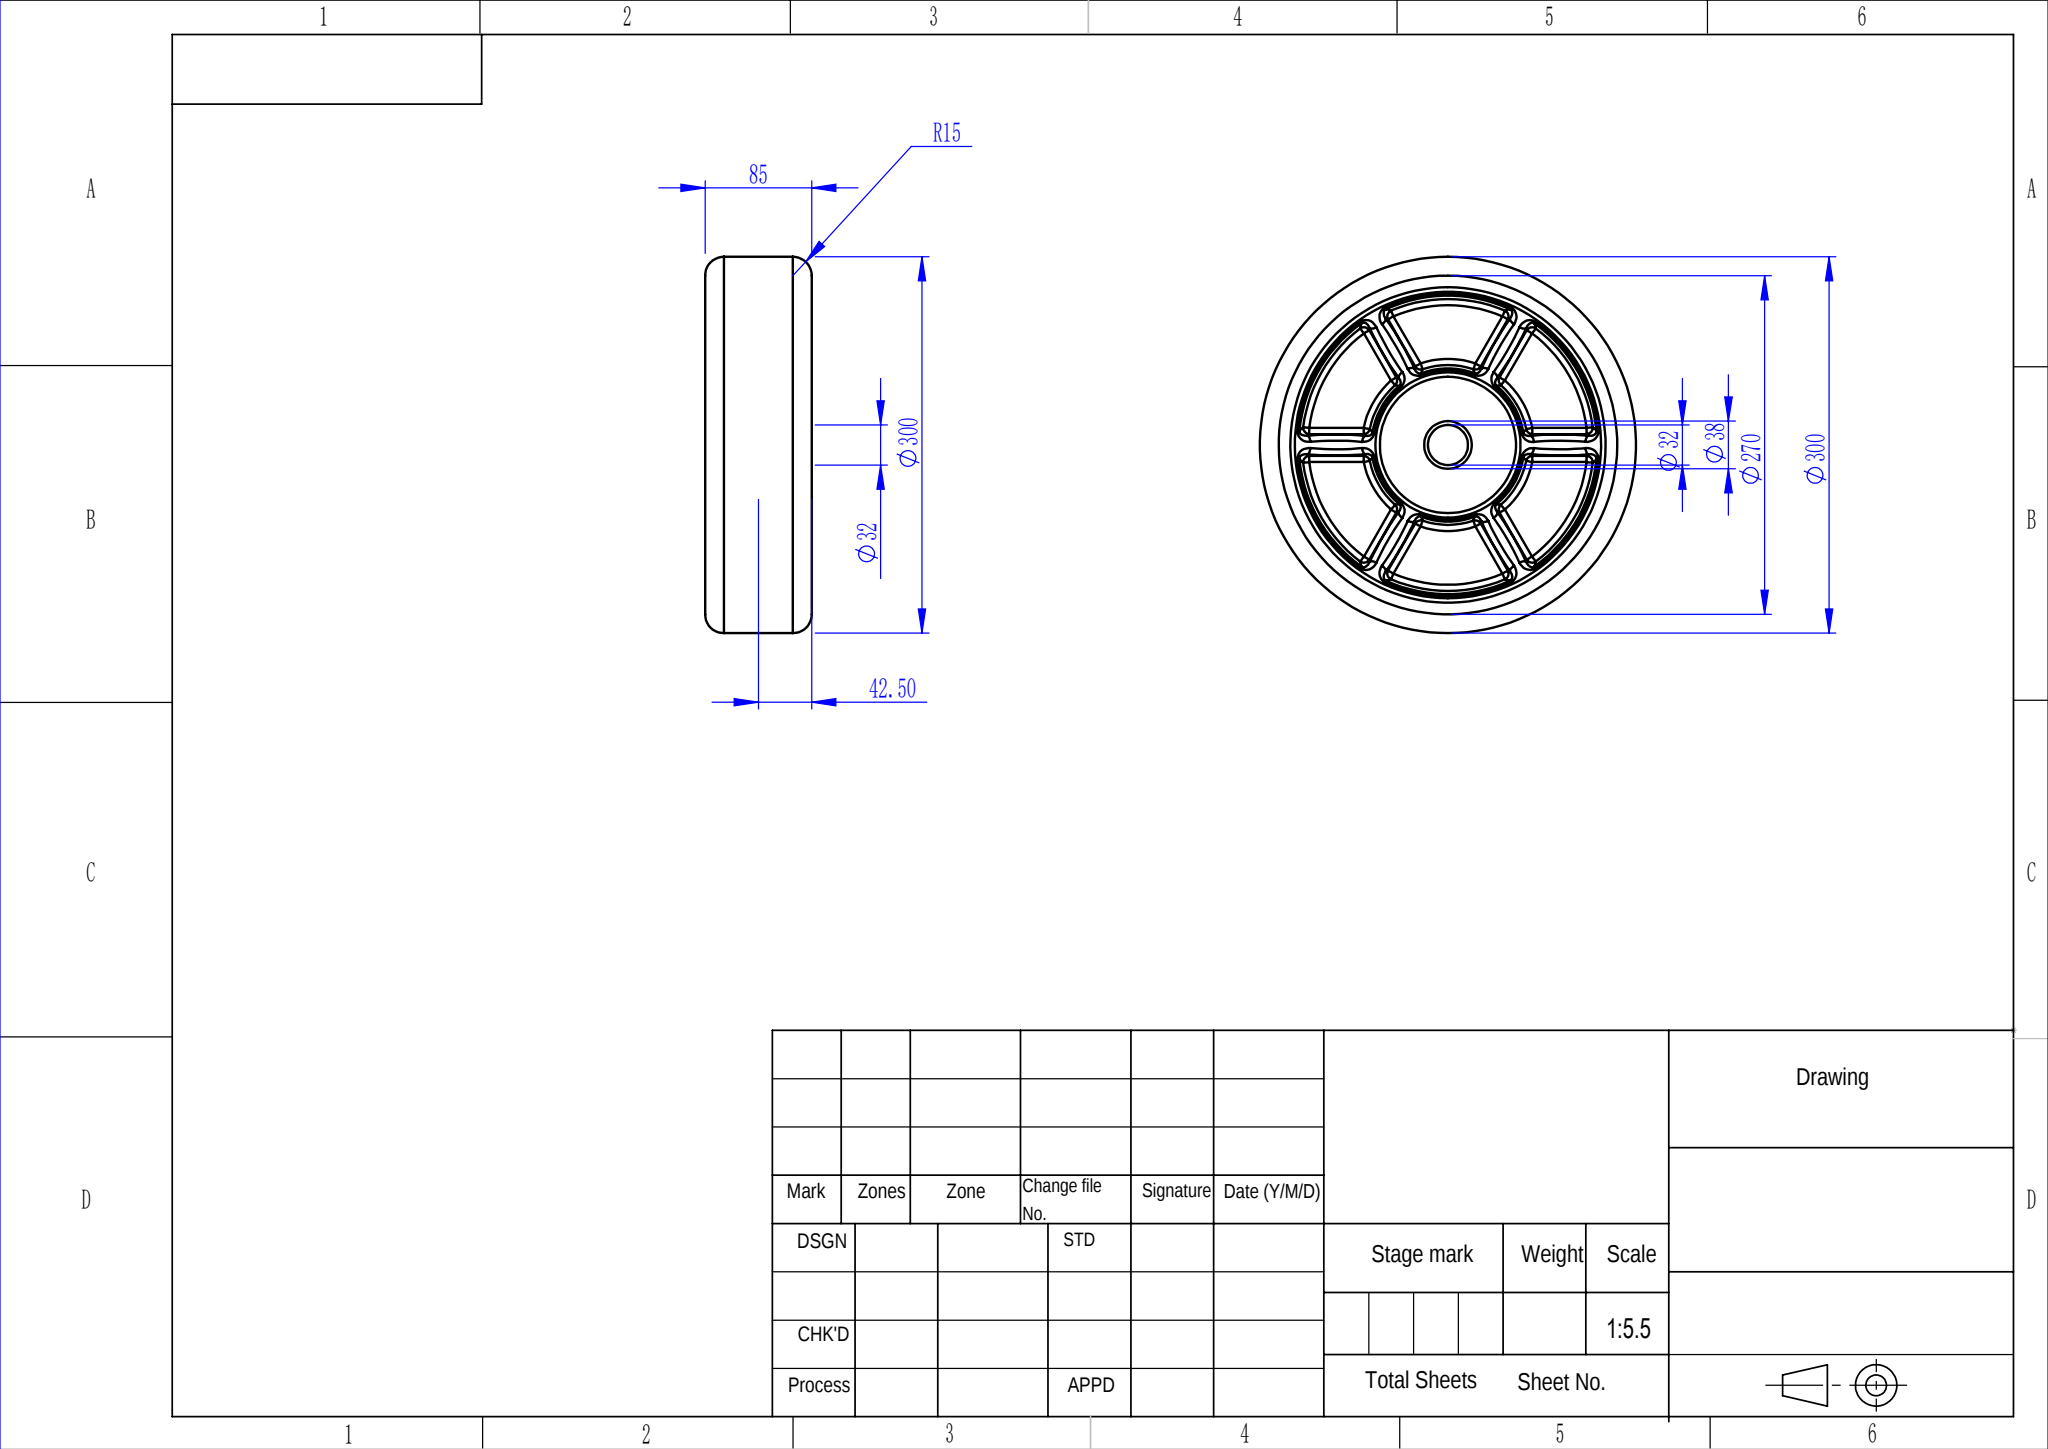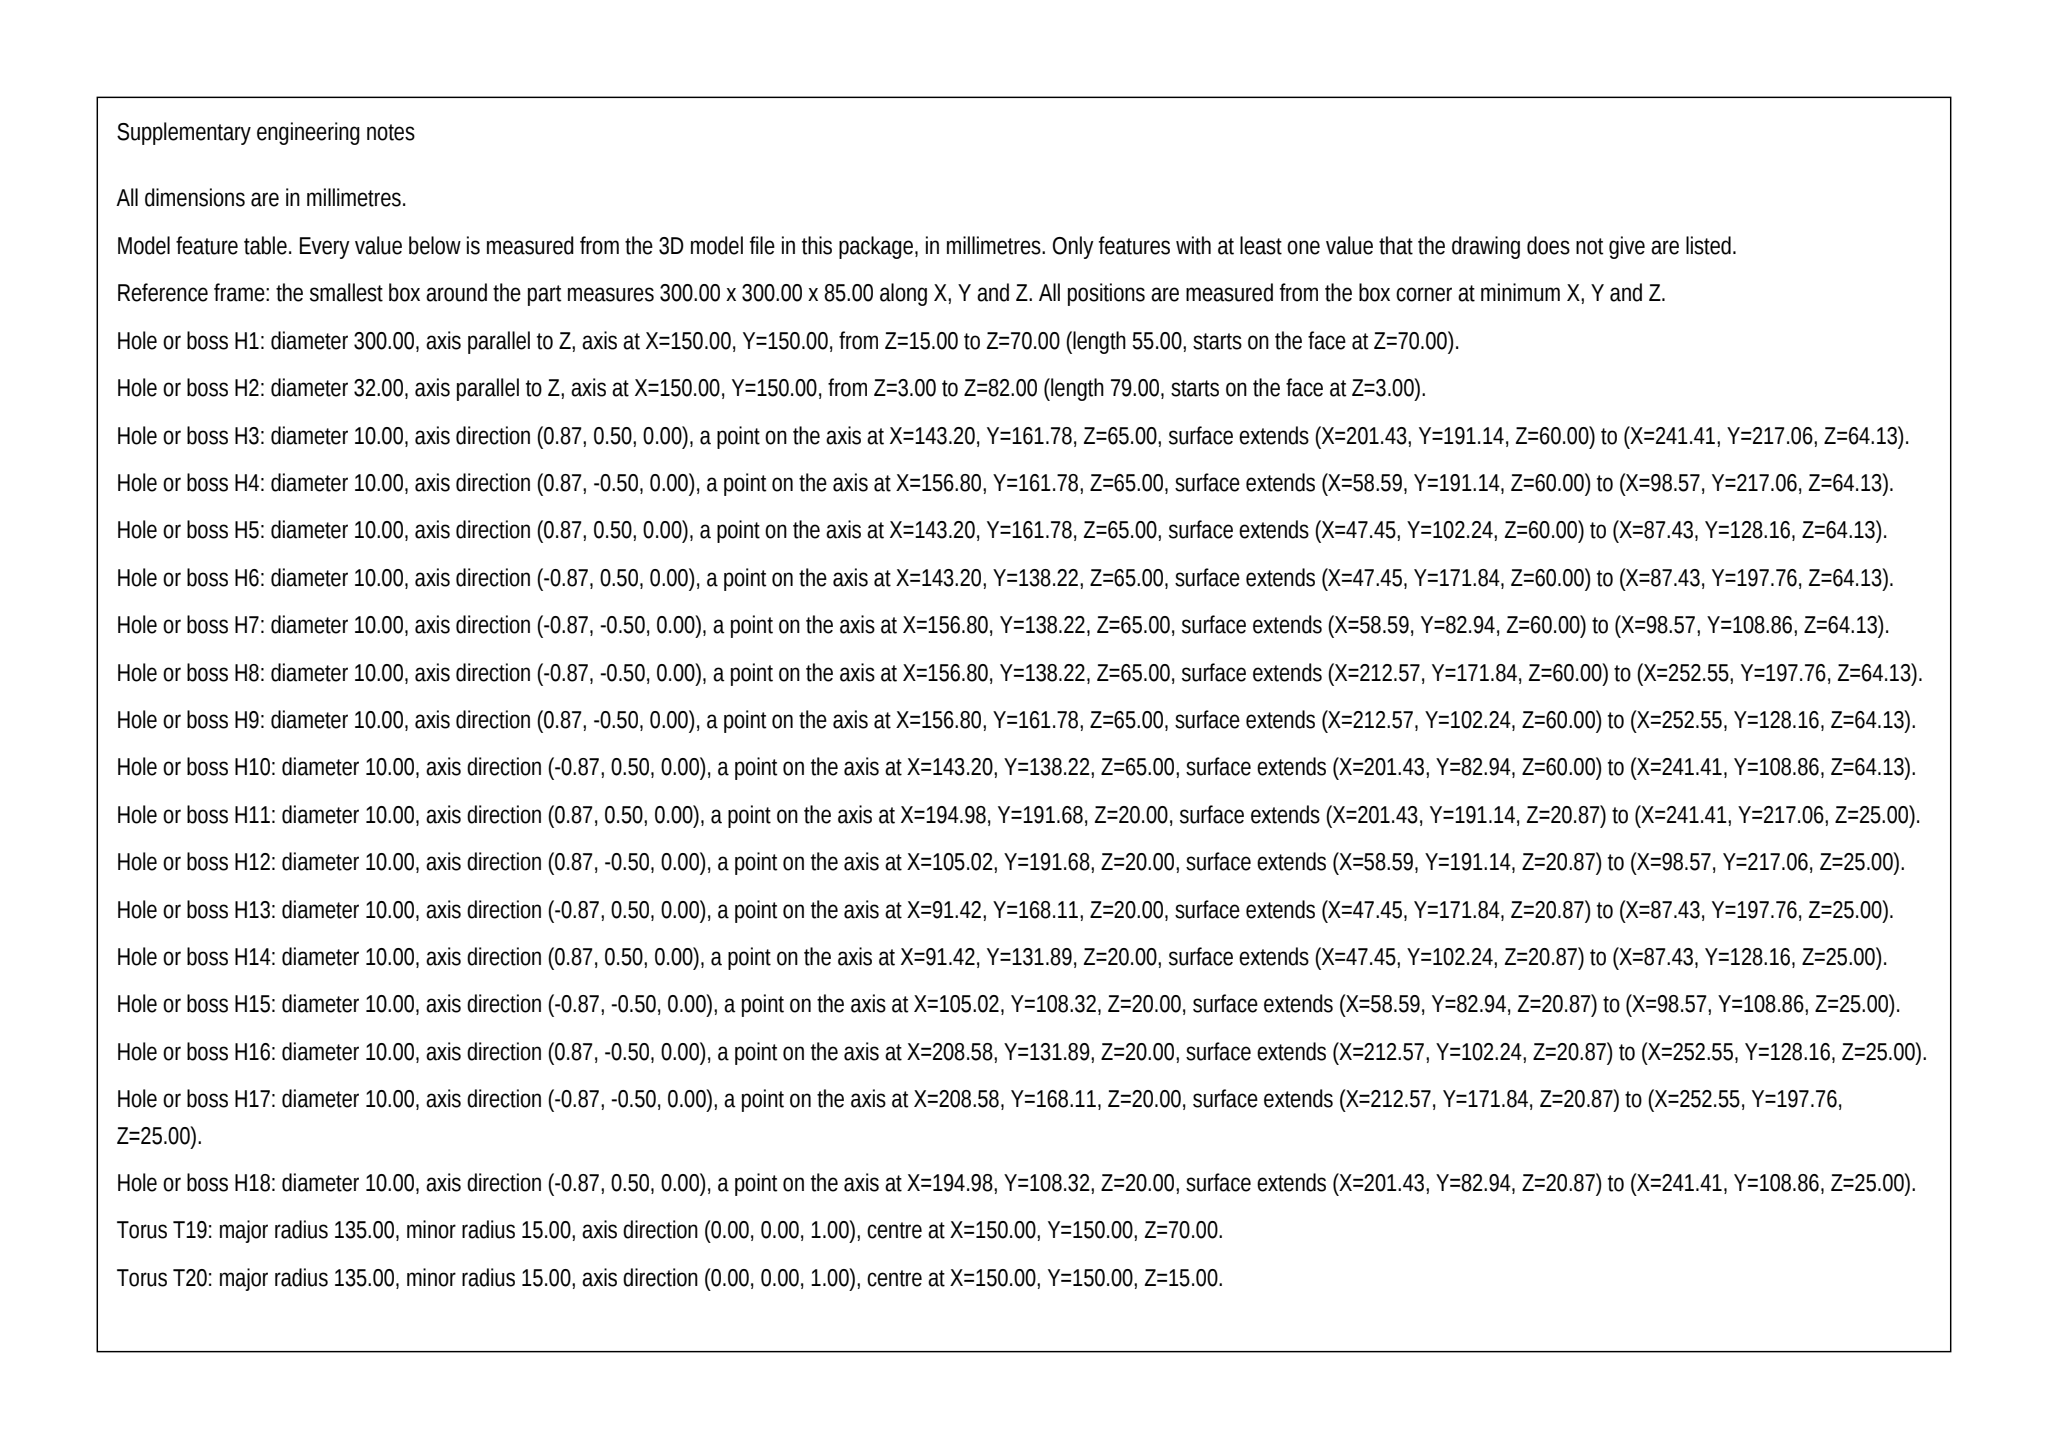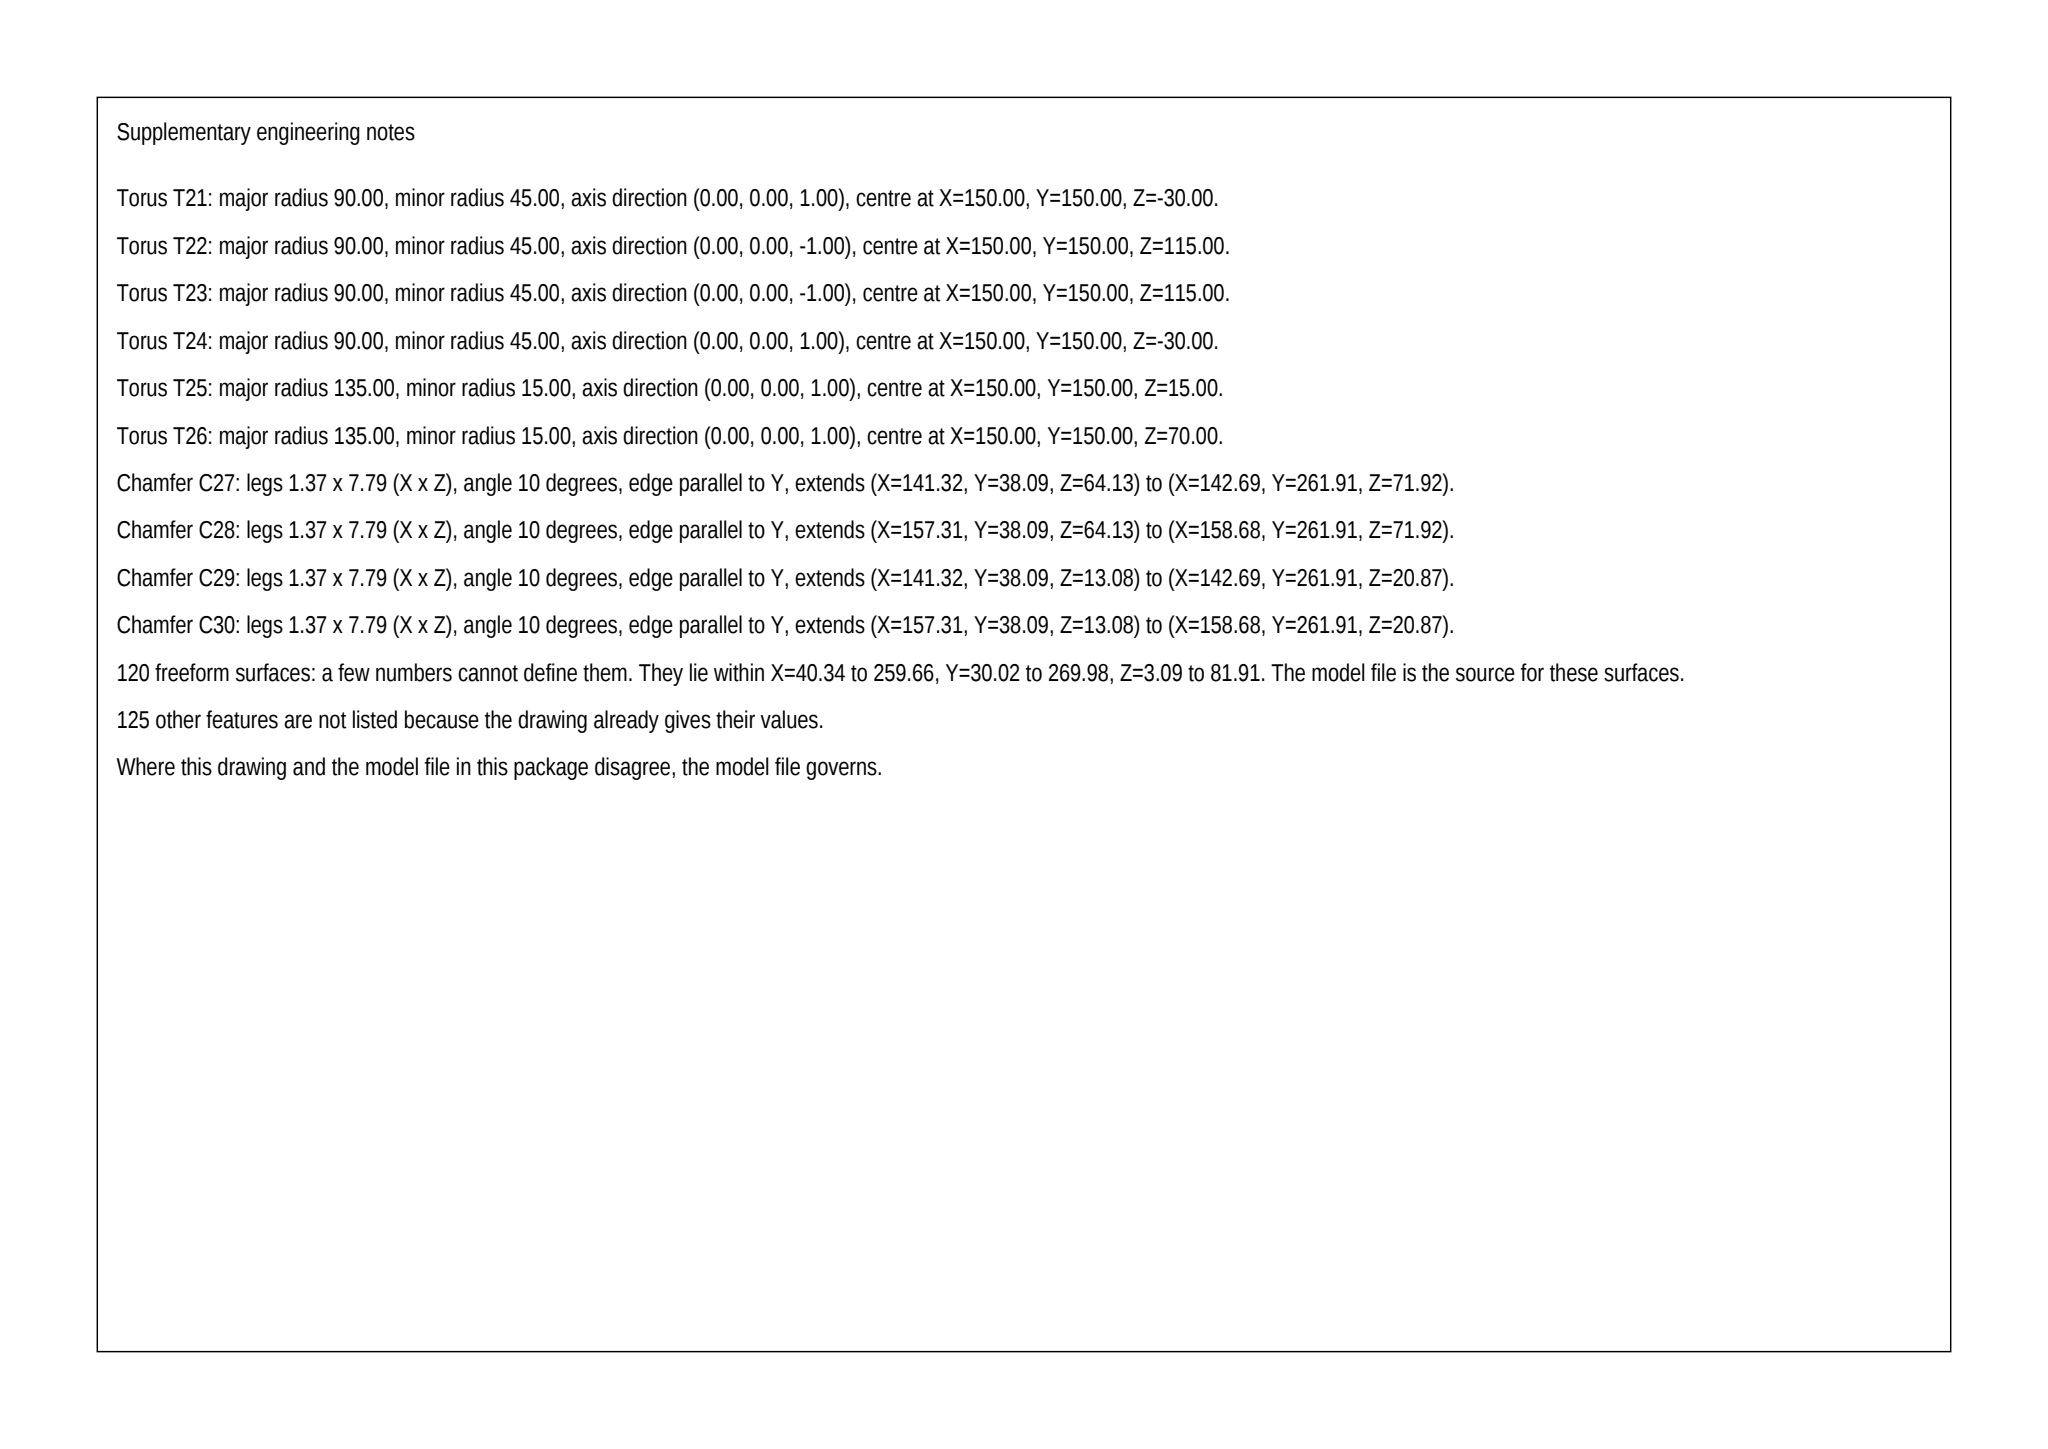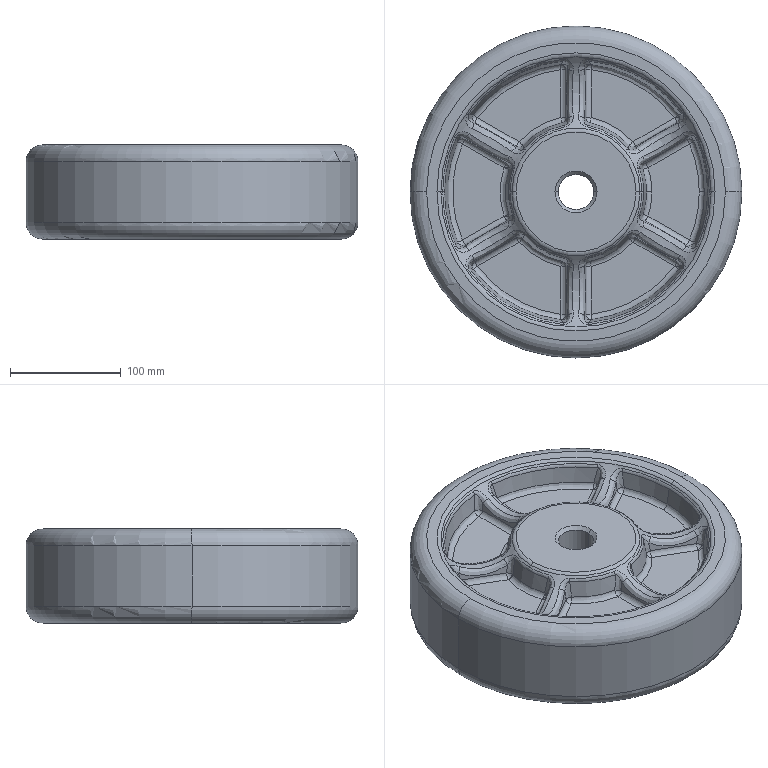Part | SolidWorks | mm | 1 solid | 348 faces | box 300 x 300 x 85 mm | volume 4407599 mm3 | spline 120 | torus 72 | sphere 56 | plane 40 | cone 32 | cylinder 28 | commonest cylinder face diameters 10 x24 32 x2 300 x2